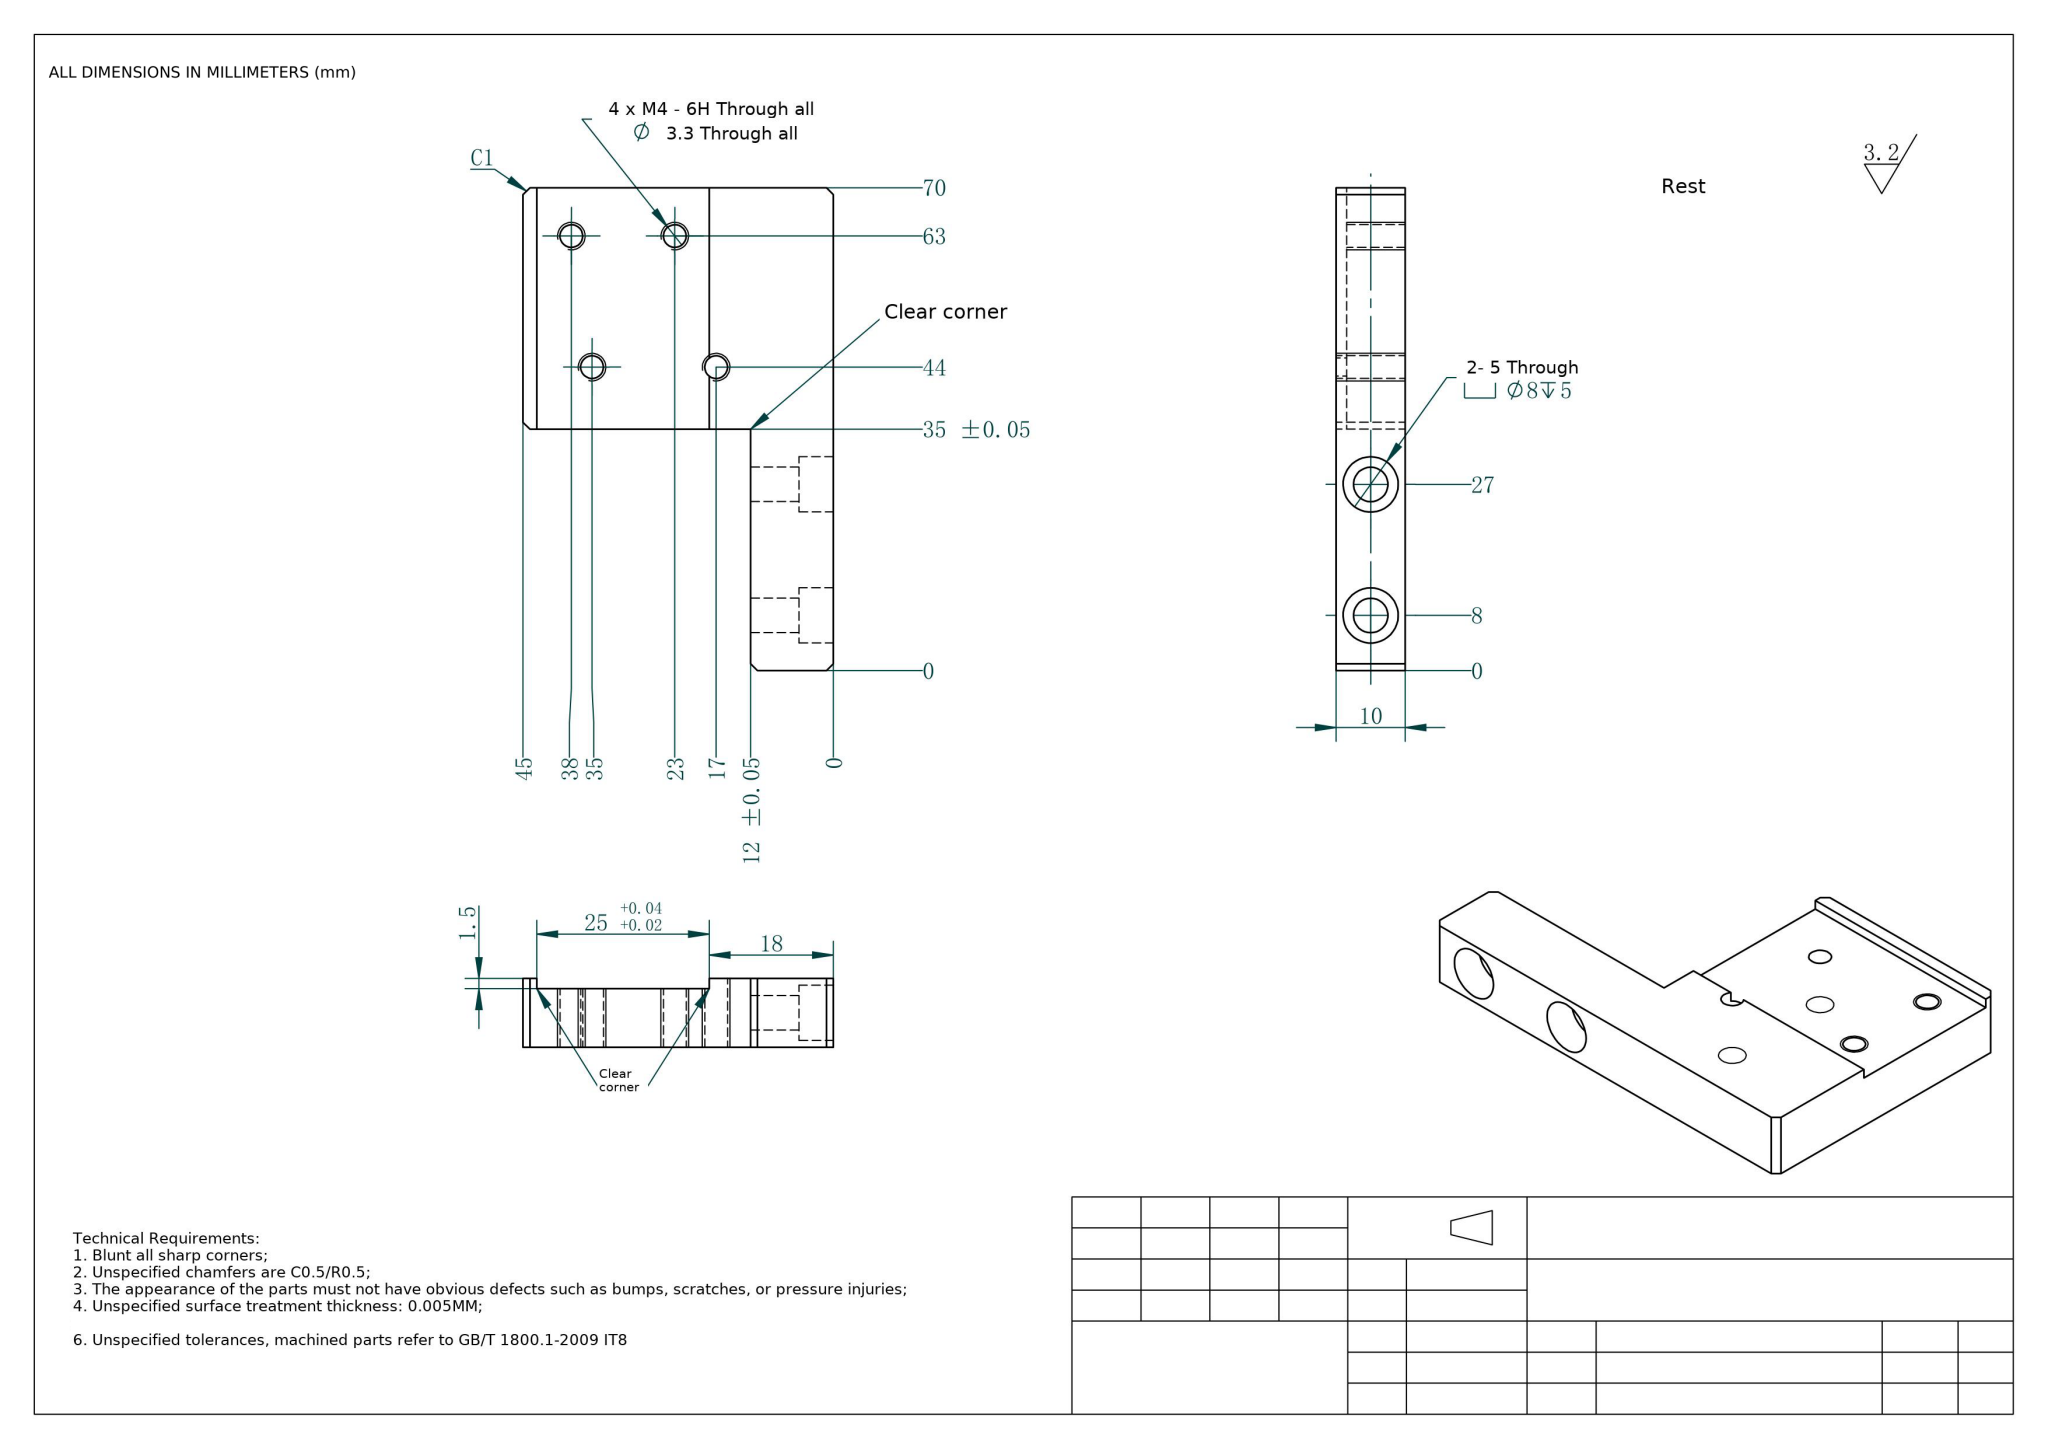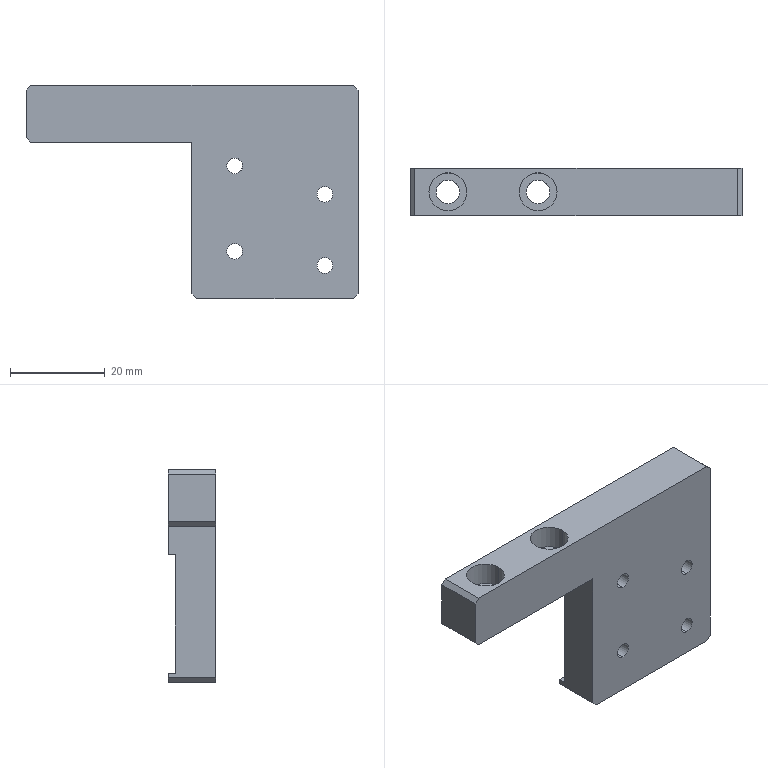Part | NX | mm | 1 solid | 36 faces | box 70 x 10 x 45 mm | volume 17533 mm3 | plane 20 | cylinder 16 | commonest cylinder face diameters 3.3 x8 8 x4 5 x4